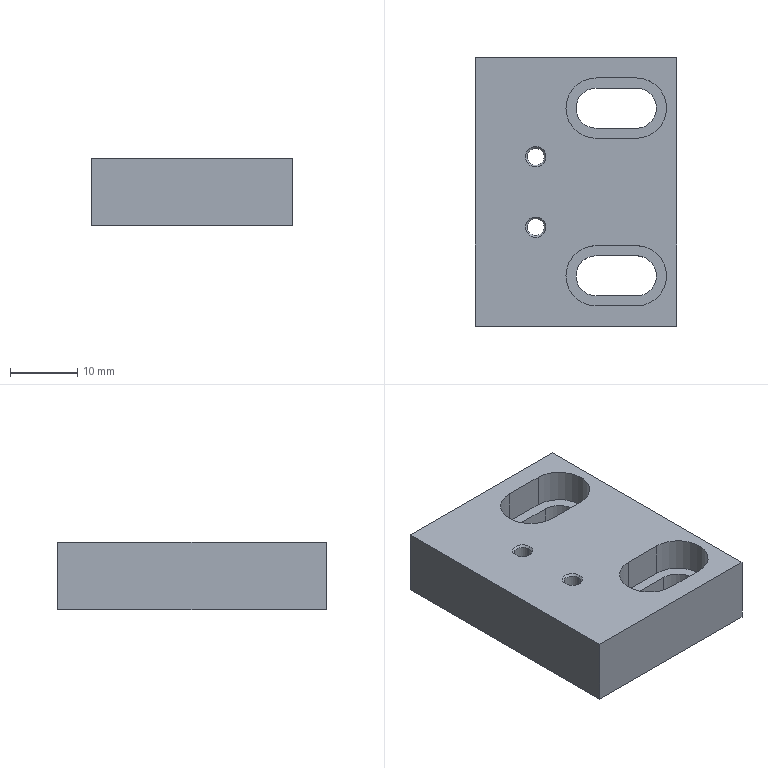Component | SolidWorks | PhotoelectricMount-1 | 1 solid | 36 faces | box 30 x 40 x 10 mm | volume 10082 mm3 | cylinder 16 | plane 16 | cone 4 | commonest cylinder face diameters 6 x6 9 x6 2.5 x4
STEP:
#1=CARTESIAN_POINT('',(-3.061,-2.53,-9.952));
#2=VERTEX_POINT('',#1);
#3=CARTESIAN_POINT('',(-3.159,-2.53,-9.952));
#4=VERTEX_POINT('',#3);
#5=CARTESIAN_POINT('',(-3.11,-2.53,-9.952));
#6=DIRECTION('',(-0.,0.,1.));
#7=DIRECTION('',(-1.,0.,0.));
#8=AXIS2_PLACEMENT_3D('',#5,#6,#7);
#9=CIRCLE('',#8,0.04921);
#10=EDGE_CURVE('',#2,#4,#9,.T.);
#11=ORIENTED_EDGE('',*,*,#10,.F.);
#12=CARTESIAN_POINT('',(-3.05,-2.53,-9.941));
#13=VERTEX_POINT('',#12);
#14=CARTESIAN_POINT('',(-3.061,-2.53,-9.952));
#15=DIRECTION('',(0.7071,-0.,0.7071));
#16=VECTOR('',#15,39.37);
#17=LINE('',#14,#16);
#18=EDGE_CURVE('',#2,#13,#17,.T.);
#19=ORIENTED_EDGE('',*,*,#18,.T.);
#20=CARTESIAN_POINT('',(-3.17,-2.53,-9.941));
#21=VERTEX_POINT('',#20);
#22=CARTESIAN_POINT('',(-3.11,-2.53,-9.941));
#23=DIRECTION('',(0.,0.,-1.));
#24=DIRECTION('',(-1.,0.,0.));
#25=AXIS2_PLACEMENT_3D('',#22,#23,#24);
#26=CIRCLE('',#25,0.06004);
#27=EDGE_CURVE('',#21,#13,#26,.T.);
#28=ORIENTED_EDGE('',*,*,#27,.F.);
#29=CARTESIAN_POINT('',(-3.159,-2.53,-9.952));
#30=DIRECTION('',(-0.7071,0.,0.7071));
#31=VECTOR('',#30,39.37);
#32=LINE('',#29,#31);
#33=EDGE_CURVE('',#4,#21,#32,.T.);
#34=ORIENTED_EDGE('',*,*,#33,.F.);
#35=EDGE_LOOP('',(#11,#19,#28,#34));
#36=FACE_OUTER_BOUND('',#35,.T.);
#37=CARTESIAN_POINT('',(-3.11,-2.53,-9.952));
#38=DIRECTION('',(-0.,0.,1.));
#39=DIRECTION('',(-1.,0.,0.));
#40=AXIS2_PLACEMENT_3D('',#37,#38,#39);
#41=CONICAL_SURFACE('',#40,0.04921,0.7854);
#42=ADVANCED_FACE('',(#36),#41,.F.);
#43=CARTESIAN_POINT('',(-3.061,-2.943,-9.952));
#44=VERTEX_POINT('',#43);
#45=CARTESIAN_POINT('',(-3.159,-2.943,-9.952));
#46=VERTEX_POINT('',#45);
#47=CARTESIAN_POINT('',(-3.11,-2.943,-9.952));
#48=DIRECTION('',(-0.,0.,1.));
#49=DIRECTION('',(-1.,0.,0.));
#50=AXIS2_PLACEMENT_3D('',#47,#48,#49);
#51=CIRCLE('',#50,0.04921);
#52=EDGE_CURVE('',#44,#46,#51,.T.);
#53=ORIENTED_EDGE('',*,*,#52,.F.);
#54=CARTESIAN_POINT('',(-3.05,-2.943,-9.941));
#55=VERTEX_POINT('',#54);
#56=CARTESIAN_POINT('',(-3.061,-2.943,-9.952));
#57=DIRECTION('',(0.7071,-0.,0.7071));
#58=VECTOR('',#57,39.37);
#59=LINE('',#56,#58);
#60=EDGE_CURVE('',#44,#55,#59,.T.);
#61=ORIENTED_EDGE('',*,*,#60,.T.);
#62=CARTESIAN_POINT('',(-3.17,-2.943,-9.941));
#63=VERTEX_POINT('',#62);
#64=CARTESIAN_POINT('',(-3.11,-2.943,-9.941));
#65=DIRECTION('',(0.,0.,-1.));
#66=DIRECTION('',(-1.,0.,0.));
#67=AXIS2_PLACEMENT_3D('',#64,#65,#66);
#68=CIRCLE('',#67,0.06004);
#69=EDGE_CURVE('',#63,#55,#68,.T.);
#70=ORIENTED_EDGE('',*,*,#69,.F.);
#71=CARTESIAN_POINT('',(-3.159,-2.943,-9.952));
#72=DIRECTION('',(-0.7071,0.,0.7071));
#73=VECTOR('',#72,39.37);
#74=LINE('',#71,#73);
#75=EDGE_CURVE('',#46,#63,#74,.T.);
#76=ORIENTED_EDGE('',*,*,#75,.F.);
#77=EDGE_LOOP('',(#53,#61,#70,#76));
#78=FACE_OUTER_BOUND('',#77,.T.);
#79=CARTESIAN_POINT('',(-3.11,-2.943,-9.952));
#80=DIRECTION('',(-0.,0.,1.));
#81=DIRECTION('',(-1.,0.,0.));
#82=AXIS2_PLACEMENT_3D('',#79,#80,#81);
#83=CONICAL_SURFACE('',#82,0.04921,0.7854);
#84=ADVANCED_FACE('',(#78),#83,.F.);
#85=CARTESIAN_POINT('',(-3.061,-2.53,-10.335));
#86=VERTEX_POINT('',#85);
#87=CARTESIAN_POINT('',(-3.159,-2.53,-10.335));
#88=VERTEX_POINT('',#87);
#89=CARTESIAN_POINT('',(-3.11,-2.53,-10.335));
#90=DIRECTION('',(-0.,0.,1.));
#91=DIRECTION('',(-1.,0.,0.));
#92=AXIS2_PLACEMENT_3D('',#89,#90,#91);
#93=CIRCLE('',#92,0.04921);
#94=EDGE_CURVE('',#86,#88,#93,.T.);
#95=ORIENTED_EDGE('',*,*,#94,.F.);
#96=CARTESIAN_POINT('',(-3.061,-2.53,-9.941));
#97=DIRECTION('',(-0.,0.,1.));
#98=VECTOR('',#97,39.37);
#99=LINE('',#96,#98);
#100=EDGE_CURVE('',#86,#2,#99,.T.);
#101=ORIENTED_EDGE('',*,*,#100,.T.);
#102=ORIENTED_EDGE('',*,*,#10,.T.);
#103=CARTESIAN_POINT('',(-3.159,-2.53,-9.941));
#104=DIRECTION('',(-0.,0.,1.));
#105=VECTOR('',#104,39.37);
#106=LINE('',#103,#105);
#107=EDGE_CURVE('',#88,#4,#106,.T.);
#108=ORIENTED_EDGE('',*,*,#107,.F.);
#109=EDGE_LOOP('',(#95,#101,#102,#108));
#110=FACE_OUTER_BOUND('',#109,.T.);
#111=CARTESIAN_POINT('',(-3.11,-2.53,-9.941));
#112=DIRECTION('',(-0.,0.,1.));
#113=DIRECTION('',(-1.,0.,0.));
#114=AXIS2_PLACEMENT_3D('',#111,#112,#113);
#115=CYLINDRICAL_SURFACE('',#114,0.04921);
#116=ADVANCED_FACE('',(#110),#115,.F.);
#117=CARTESIAN_POINT('',(-3.061,-2.943,-10.335));
#118=VERTEX_POINT('',#117);
#119=CARTESIAN_POINT('',(-3.159,-2.943,-10.335));
#120=VERTEX_POINT('',#119);
#121=CARTESIAN_POINT('',(-3.11,-2.943,-10.335));
#122=DIRECTION('',(-0.,0.,1.));
#123=DIRECTION('',(-1.,0.,0.));
#124=AXIS2_PLACEMENT_3D('',#121,#122,#123);
#125=CIRCLE('',#124,0.04921);
#126=EDGE_CURVE('',#118,#120,#125,.T.);
#127=ORIENTED_EDGE('',*,*,#126,.F.);
#128=CARTESIAN_POINT('',(-3.061,-2.943,-9.941));
#129=DIRECTION('',(-0.,0.,1.));
#130=VECTOR('',#129,39.37);
#131=LINE('',#128,#130);
#132=EDGE_CURVE('',#118,#44,#131,.T.);
#133=ORIENTED_EDGE('',*,*,#132,.T.);
#134=ORIENTED_EDGE('',*,*,#52,.T.);
#135=CARTESIAN_POINT('',(-3.159,-2.943,-9.941));
#136=DIRECTION('',(-0.,0.,1.));
#137=VECTOR('',#136,39.37);
#138=LINE('',#135,#137);
#139=EDGE_CURVE('',#120,#46,#138,.T.);
#140=ORIENTED_EDGE('',*,*,#139,.F.);
#141=EDGE_LOOP('',(#127,#133,#134,#140));
#142=FACE_OUTER_BOUND('',#141,.T.);
#143=CARTESIAN_POINT('',(-3.11,-2.943,-9.941));
#144=DIRECTION('',(-0.,0.,1.));
#145=DIRECTION('',(-1.,0.,0.));
#146=AXIS2_PLACEMENT_3D('',#143,#144,#145);
#147=CYLINDRICAL_SURFACE('',#146,0.04921);
#148=ADVANCED_FACE('',(#142),#147,.F.);
#149=CARTESIAN_POINT('',(-2.52,-2.362,-10.138));
#150=VERTEX_POINT('',#149);
#151=CARTESIAN_POINT('',(-2.402,-2.244,-10.138));
#152=VERTEX_POINT('',#151);
#153=CARTESIAN_POINT('',(-2.52,-2.244,-10.138));
#154=DIRECTION('',(-0.,0.,1.));
#155=DIRECTION('',(-1.,0.,0.));
#156=AXIS2_PLACEMENT_3D('',#153,#154,#155);
#157=CIRCLE('',#156,0.1181);
#158=EDGE_CURVE('',#150,#152,#157,.T.);
#159=ORIENTED_EDGE('',*,*,#158,.T.);
#160=CARTESIAN_POINT('',(-2.402,-2.244,-10.335));
#161=VERTEX_POINT('',#160);
#162=CARTESIAN_POINT('',(-2.402,-2.244,-9.941));
#163=DIRECTION('',(0.,0.,-1.));
#164=VECTOR('',#163,39.37);
#165=LINE('',#162,#164);
#166=EDGE_CURVE('',#152,#161,#165,.T.);
#167=ORIENTED_EDGE('',*,*,#166,.T.);
#168=CARTESIAN_POINT('',(-2.52,-2.362,-10.335));
#169=VERTEX_POINT('',#168);
#170=CARTESIAN_POINT('',(-2.52,-2.244,-10.335));
#171=DIRECTION('',(0.,0.,-1.));
#172=DIRECTION('',(1.,0.,0.));
#173=AXIS2_PLACEMENT_3D('',#170,#171,#172);
#174=CIRCLE('',#173,0.1181);
#175=EDGE_CURVE('',#161,#169,#174,.T.);
#176=ORIENTED_EDGE('',*,*,#175,.T.);
#177=CARTESIAN_POINT('',(-2.52,-2.362,-9.941));
#178=DIRECTION('',(0.,0.,-1.));
#179=VECTOR('',#178,39.37);
#180=LINE('',#177,#179);
#181=EDGE_CURVE('',#150,#169,#180,.T.);
#182=ORIENTED_EDGE('',*,*,#181,.F.);
#183=EDGE_LOOP('',(#159,#167,#176,#182));
#184=FACE_OUTER_BOUND('',#183,.T.);
#185=CARTESIAN_POINT('',(-2.52,-2.244,-9.941));
#186=DIRECTION('',(0.,0.,-1.));
#187=DIRECTION('',(1.,0.,0.));
#188=AXIS2_PLACEMENT_3D('',#185,#186,#187);
#189=CYLINDRICAL_SURFACE('',#188,0.1181);
#190=ADVANCED_FACE('',(#184),#189,.F.);
#191=CARTESIAN_POINT('',(-2.933,-2.244,-10.138));
#192=VERTEX_POINT('',#191);
#193=CARTESIAN_POINT('',(-2.756,-2.421,-10.138));
#194=VERTEX_POINT('',#193);
#195=CARTESIAN_POINT('',(-2.756,-2.244,-10.138));
#196=DIRECTION('',(-0.,0.,1.));
#197=DIRECTION('',(-1.,0.,0.));
#198=AXIS2_PLACEMENT_3D('',#195,#196,#197);
#199=CIRCLE('',#198,0.1772);
#200=EDGE_CURVE('',#192,#194,#199,.T.);
#201=ORIENTED_EDGE('',*,*,#200,.F.);
#202=CARTESIAN_POINT('',(-2.933,-2.244,-9.941));
#203=VERTEX_POINT('',#202);
#204=CARTESIAN_POINT('',(-2.933,-2.244,-10.138));
#205=DIRECTION('',(-0.,0.,1.));
#206=VECTOR('',#205,39.37);
#207=LINE('',#204,#206);
#208=EDGE_CURVE('',#192,#203,#207,.T.);
#209=ORIENTED_EDGE('',*,*,#208,.T.);
#210=CARTESIAN_POINT('',(-2.756,-2.421,-9.941));
#211=VERTEX_POINT('',#210);
#212=CARTESIAN_POINT('',(-2.756,-2.244,-9.941));
#213=DIRECTION('',(-0.,0.,1.));
#214=DIRECTION('',(-1.,0.,0.));
#215=AXIS2_PLACEMENT_3D('',#212,#213,#214);
#216=CIRCLE('',#215,0.1772);
#217=EDGE_CURVE('',#203,#211,#216,.T.);
#218=ORIENTED_EDGE('',*,*,#217,.T.);
#219=CARTESIAN_POINT('',(-2.756,-2.421,-10.138));
#220=DIRECTION('',(-0.,0.,1.));
#221=VECTOR('',#220,39.37);
#222=LINE('',#219,#221);
#223=EDGE_CURVE('',#194,#211,#222,.T.);
#224=ORIENTED_EDGE('',*,*,#223,.F.);
#225=EDGE_LOOP('',(#201,#209,#218,#224));
#226=FACE_OUTER_BOUND('',#225,.T.);
#227=CARTESIAN_POINT('',(-2.756,-2.244,-10.138));
#228=DIRECTION('',(-0.,0.,1.));
#229=DIRECTION('',(-1.,0.,0.));
#230=AXIS2_PLACEMENT_3D('',#227,#228,#229);
#231=CYLINDRICAL_SURFACE('',#230,0.1772);
#232=ADVANCED_FACE('',(#226),#231,.F.);
#233=CARTESIAN_POINT('',(-2.52,-3.346,-10.138));
#234=VERTEX_POINT('',#233);
#235=CARTESIAN_POINT('',(-2.402,-3.228,-10.138));
#236=VERTEX_POINT('',#235);
#237=CARTESIAN_POINT('',(-2.52,-3.228,-10.138));
#238=DIRECTION('',(-0.,0.,1.));
#239=DIRECTION('',(-1.,0.,0.));
#240=AXIS2_PLACEMENT_3D('',#237,#238,#239);
#241=CIRCLE('',#240,0.1181);
#242=EDGE_CURVE('',#234,#236,#241,.T.);
#243=ORIENTED_EDGE('',*,*,#242,.T.);
#244=CARTESIAN_POINT('',(-2.402,-3.228,-10.335));
#245=VERTEX_POINT('',#244);
#246=CARTESIAN_POINT('',(-2.402,-3.228,-9.941));
#247=DIRECTION('',(0.,0.,-1.));
#248=VECTOR('',#247,39.37);
#249=LINE('',#246,#248);
#250=EDGE_CURVE('',#236,#245,#249,.T.);
#251=ORIENTED_EDGE('',*,*,#250,.T.);
#252=CARTESIAN_POINT('',(-2.52,-3.346,-10.335));
#253=VERTEX_POINT('',#252);
#254=CARTESIAN_POINT('',(-2.52,-3.228,-10.335));
#255=DIRECTION('',(0.,0.,-1.));
#256=DIRECTION('',(1.,0.,0.));
#257=AXIS2_PLACEMENT_3D('',#254,#255,#256);
#258=CIRCLE('',#257,0.1181);
#259=EDGE_CURVE('',#245,#253,#258,.T.);
#260=ORIENTED_EDGE('',*,*,#259,.T.);
#261=CARTESIAN_POINT('',(-2.52,-3.346,-9.941));
#262=DIRECTION('',(0.,0.,-1.));
#263=VECTOR('',#262,39.37);
#264=LINE('',#261,#263);
#265=EDGE_CURVE('',#234,#253,#264,.T.);
#266=ORIENTED_EDGE('',*,*,#265,.F.);
#267=EDGE_LOOP('',(#243,#251,#260,#266));
#268=FACE_OUTER_BOUND('',#267,.T.);
#269=CARTESIAN_POINT('',(-2.52,-3.228,-9.941));
#270=DIRECTION('',(0.,0.,-1.));
#271=DIRECTION('',(1.,0.,0.));
#272=AXIS2_PLACEMENT_3D('',#269,#270,#271);
#273=CYLINDRICAL_SURFACE('',#272,0.1181);
#274=ADVANCED_FACE('',(#268),#273,.F.);
#275=CARTESIAN_POINT('',(-2.933,-3.228,-10.138));
#276=VERTEX_POINT('',#275);
#277=CARTESIAN_POINT('',(-2.756,-3.406,-10.138));
#278=VERTEX_POINT('',#277);
#279=CARTESIAN_POINT('',(-2.756,-3.228,-10.138));
#280=DIRECTION('',(-0.,0.,1.));
#281=DIRECTION('',(-1.,0.,0.));
#282=AXIS2_PLACEMENT_3D('',#279,#280,#281);
#283=CIRCLE('',#282,0.1772);
#284=EDGE_CURVE('',#276,#278,#283,.T.);
#285=ORIENTED_EDGE('',*,*,#284,.F.);
#286=CARTESIAN_POINT('',(-2.933,-3.228,-9.941));
#287=VERTEX_POINT('',#286);
#288=CARTESIAN_POINT('',(-2.933,-3.228,-10.138));
#289=DIRECTION('',(-0.,0.,1.));
#290=VECTOR('',#289,39.37);
#291=LINE('',#288,#290);
#292=EDGE_CURVE('',#276,#287,#291,.T.);
#293=ORIENTED_EDGE('',*,*,#292,.T.);
#294=CARTESIAN_POINT('',(-2.756,-3.406,-9.941));
#295=VERTEX_POINT('',#294);
#296=CARTESIAN_POINT('',(-2.756,-3.228,-9.941));
#297=DIRECTION('',(-0.,0.,1.));
#298=DIRECTION('',(-1.,0.,0.));
#299=AXIS2_PLACEMENT_3D('',#296,#297,#298);
#300=CIRCLE('',#299,0.1772);
#301=EDGE_CURVE('',#287,#295,#300,.T.);
#302=ORIENTED_EDGE('',*,*,#301,.T.);
#303=CARTESIAN_POINT('',(-2.756,-3.406,-10.138));
#304=DIRECTION('',(-0.,0.,1.));
#305=VECTOR('',#304,39.37);
#306=LINE('',#303,#305);
#307=EDGE_CURVE('',#278,#295,#306,.T.);
#308=ORIENTED_EDGE('',*,*,#307,.F.);
#309=EDGE_LOOP('',(#285,#293,#302,#308));
#310=FACE_OUTER_BOUND('',#309,.T.);
#311=CARTESIAN_POINT('',(-2.756,-3.228,-10.138));
#312=DIRECTION('',(-0.,0.,1.));
#313=DIRECTION('',(-1.,0.,0.));
#314=AXIS2_PLACEMENT_3D('',#311,#312,#313);
#315=CYLINDRICAL_SURFACE('',#314,0.1772);
#316=ADVANCED_FACE('',(#310),#315,.F.);
#317=CARTESIAN_POINT('',(-3.465,-3.524,-9.941));
#318=VERTEX_POINT('',#317);
#319=CARTESIAN_POINT('',(-2.283,-3.524,-9.941));
#320=VERTEX_POINT('',#319);
#321=CARTESIAN_POINT('',(-3.465,-3.524,-9.941));
#322=DIRECTION('',(1.,-0.,0.));
#323=VECTOR('',#322,39.37);
#324=LINE('',#321,#323);
#325=EDGE_CURVE('',#318,#320,#324,.T.);
#326=ORIENTED_EDGE('',*,*,#325,.F.);
#327=CARTESIAN_POINT('',(-3.465,-3.524,-10.335));
#328=VERTEX_POINT('',#327);
#329=CARTESIAN_POINT('',(-3.465,-3.524,-10.335));
#330=DIRECTION('',(-0.,0.,1.));
#331=VECTOR('',#330,39.37);
#332=LINE('',#329,#331);
#333=EDGE_CURVE('',#328,#318,#332,.T.);
#334=ORIENTED_EDGE('',*,*,#333,.F.);
#335=CARTESIAN_POINT('',(-2.283,-3.524,-10.335));
#336=VERTEX_POINT('',#335);
#337=CARTESIAN_POINT('',(-3.465,-3.524,-10.335));
#338=DIRECTION('',(1.,-0.,0.));
#339=VECTOR('',#338,39.37);
#340=LINE('',#337,#339);
#341=EDGE_CURVE('',#328,#336,#340,.T.);
#342=ORIENTED_EDGE('',*,*,#341,.T.);
#343=CARTESIAN_POINT('',(-2.283,-3.524,-10.335));
#344=DIRECTION('',(-0.,0.,1.));
#345=VECTOR('',#344,39.37);
#346=LINE('',#343,#345);
#347=EDGE_CURVE('',#336,#320,#346,.T.);
#348=ORIENTED_EDGE('',*,*,#347,.T.);
#349=EDGE_LOOP('',(#326,#334,#342,#348));
#350=FACE_OUTER_BOUND('',#349,.T.);
#351=CARTESIAN_POINT('',(-3.465,-3.524,-10.335));
#352=DIRECTION('',(-0.,-1.,-0.));
#353=DIRECTION('',(-0.,0.,1.));
#354=AXIS2_PLACEMENT_3D('',#351,#352,#353);
#355=PLANE('',#354);
#356=ADVANCED_FACE('',(#350),#355,.T.);
#357=CARTESIAN_POINT('',(-3.465,-1.949,-9.941));
#358=VERTEX_POINT('',#357);
#359=CARTESIAN_POINT('',(-3.465,-1.949,-9.941));
#360=DIRECTION('',(-0.,-1.,-0.));
#361=VECTOR('',#360,39.37);
#362=LINE('',#359,#361);
#363=EDGE_CURVE('',#358,#318,#362,.T.);
#364=ORIENTED_EDGE('',*,*,#363,.F.);
#365=CARTESIAN_POINT('',(-3.465,-1.949,-10.335));
#366=VERTEX_POINT('',#365);
#367=CARTESIAN_POINT('',(-3.465,-1.949,-10.335));
#368=DIRECTION('',(-0.,0.,1.));
#369=VECTOR('',#368,39.37);
#370=LINE('',#367,#369);
#371=EDGE_CURVE('',#366,#358,#370,.T.);
#372=ORIENTED_EDGE('',*,*,#371,.F.);
#373=CARTESIAN_POINT('',(-3.465,-1.949,-10.335));
#374=DIRECTION('',(-0.,-1.,-0.));
#375=VECTOR('',#374,39.37);
#376=LINE('',#373,#375);
#377=EDGE_CURVE('',#366,#328,#376,.T.);
#378=ORIENTED_EDGE('',*,*,#377,.T.);
#379=ORIENTED_EDGE('',*,*,#333,.T.);
#380=EDGE_LOOP('',(#364,#372,#378,#379));
#381=FACE_OUTER_BOUND('',#380,.T.);
#382=CARTESIAN_POINT('',(-3.465,-1.949,-10.335));
#383=DIRECTION('',(-1.,0.,-0.));
#384=DIRECTION('',(0.,0.,-1.));
#385=AXIS2_PLACEMENT_3D('',#382,#383,#384);
#386=PLANE('',#385);
#387=ADVANCED_FACE('',(#381),#386,.T.);
#388=CARTESIAN_POINT('',(-2.283,-1.949,-9.941));
#389=VERTEX_POINT('',#388);
#390=CARTESIAN_POINT('',(-2.283,-1.949,-9.941));
#391=DIRECTION('',(-1.,0.,-0.));
#392=VECTOR('',#391,39.37);
#393=LINE('',#390,#392);
#394=EDGE_CURVE('',#389,#358,#393,.T.);
#395=ORIENTED_EDGE('',*,*,#394,.F.);
#396=CARTESIAN_POINT('',(-2.283,-1.949,-10.335));
#397=VERTEX_POINT('',#396);
#398=CARTESIAN_POINT('',(-2.283,-1.949,-10.335));
#399=DIRECTION('',(-0.,0.,1.));
#400=VECTOR('',#399,39.37);
#401=LINE('',#398,#400);
#402=EDGE_CURVE('',#397,#389,#401,.T.);
#403=ORIENTED_EDGE('',*,*,#402,.F.);
#404=CARTESIAN_POINT('',(-2.283,-1.949,-10.335));
#405=DIRECTION('',(-1.,0.,-0.));
#406=VECTOR('',#405,39.37);
#407=LINE('',#404,#406);
#408=EDGE_CURVE('',#397,#366,#407,.T.);
#409=ORIENTED_EDGE('',*,*,#408,.T.);
#410=ORIENTED_EDGE('',*,*,#371,.T.);
#411=EDGE_LOOP('',(#395,#403,#409,#410));
#412=FACE_OUTER_BOUND('',#411,.T.);
#413=CARTESIAN_POINT('',(-2.283,-1.949,-10.335));
#414=DIRECTION('',(0.,1.,0.));
#415=DIRECTION('',(0.,0.,-1.));
#416=AXIS2_PLACEMENT_3D('',#413,#414,#415);
#417=PLANE('',#416);
#418=ADVANCED_FACE('',(#412),#417,.T.);
#419=CARTESIAN_POINT('',(-2.283,-3.524,-9.941));
#420=DIRECTION('',(0.,1.,0.));
#421=VECTOR('',#420,39.37);
#422=LINE('',#419,#421);
#423=EDGE_CURVE('',#320,#389,#422,.T.);
#424=ORIENTED_EDGE('',*,*,#423,.F.);
#425=ORIENTED_EDGE('',*,*,#347,.F.);
#426=CARTESIAN_POINT('',(-2.283,-3.524,-10.335));
#427=DIRECTION('',(0.,1.,0.));
#428=VECTOR('',#427,39.37);
#429=LINE('',#426,#428);
#430=EDGE_CURVE('',#336,#397,#429,.T.);
#431=ORIENTED_EDGE('',*,*,#430,.T.);
#432=ORIENTED_EDGE('',*,*,#402,.T.);
#433=EDGE_LOOP('',(#424,#425,#431,#432));
#434=FACE_OUTER_BOUND('',#433,.T.);
#435=CARTESIAN_POINT('',(-2.283,-3.524,-10.335));
#436=DIRECTION('',(1.,-0.,0.));
#437=DIRECTION('',(-0.,0.,1.));
#438=AXIS2_PLACEMENT_3D('',#435,#436,#437);
#439=PLANE('',#438);
#440=ADVANCED_FACE('',(#434),#439,.T.);
#441=CARTESIAN_POINT('',(-3.11,-2.53,-10.335));
#442=DIRECTION('',(-0.,0.,1.));
#443=DIRECTION('',(-1.,0.,0.));
#444=AXIS2_PLACEMENT_3D('',#441,#442,#443);
#445=CIRCLE('',#444,0.04921);
#446=EDGE_CURVE('',#88,#86,#445,.T.);
#447=ORIENTED_EDGE('',*,*,#446,.T.);
#448=ORIENTED_EDGE('',*,*,#94,.T.);
#449=EDGE_LOOP('',(#447,#448));
#450=FACE_BOUND('',#449,.T.);
#451=CARTESIAN_POINT('',(-3.11,-2.943,-10.335));
#452=DIRECTION('',(-0.,0.,1.));
#453=DIRECTION('',(-1.,0.,0.));
#454=AXIS2_PLACEMENT_3D('',#451,#452,#453);
#455=CIRCLE('',#454,0.04921);
#456=EDGE_CURVE('',#120,#118,#455,.T.);
#457=ORIENTED_EDGE('',*,*,#456,.T.);
#458=ORIENTED_EDGE('',*,*,#126,.T.);
#459=EDGE_LOOP('',(#457,#458));
#460=FACE_BOUND('',#459,.T.);
#461=CARTESIAN_POINT('',(-2.756,-2.362,-10.335));
#462=VERTEX_POINT('',#461);
#463=CARTESIAN_POINT('',(-2.52,-2.362,-10.335));
#464=DIRECTION('',(-1.,0.,-0.));
#465=VECTOR('',#464,39.37);
#466=LINE('',#463,#465);
#467=EDGE_CURVE('',#169,#462,#466,.T.);
#468=ORIENTED_EDGE('',*,*,#467,.F.);
#469=ORIENTED_EDGE('',*,*,#175,.F.);
#470=CARTESIAN_POINT('',(-2.52,-2.126,-10.335));
#471=VERTEX_POINT('',#470);
#472=CARTESIAN_POINT('',(-2.52,-2.244,-10.335));
#473=DIRECTION('',(0.,0.,-1.));
#474=DIRECTION('',(1.,0.,0.));
#475=AXIS2_PLACEMENT_3D('',#472,#473,#474);
#476=CIRCLE('',#475,0.1181);
#477=EDGE_CURVE('',#471,#161,#476,.T.);
#478=ORIENTED_EDGE('',*,*,#477,.F.);
#479=CARTESIAN_POINT('',(-2.756,-2.126,-10.335));
#480=VERTEX_POINT('',#479);
#481=CARTESIAN_POINT('',(-2.756,-2.126,-10.335));
#482=DIRECTION('',(1.,-0.,0.));
#483=VECTOR('',#482,39.37);
#484=LINE('',#481,#483);
#485=EDGE_CURVE('',#480,#471,#484,.T.);
#486=ORIENTED_EDGE('',*,*,#485,.F.);
#487=CARTESIAN_POINT('',(-2.756,-2.244,-10.335));
#488=DIRECTION('',(0.,0.,-1.));
#489=DIRECTION('',(1.,0.,0.));
#490=AXIS2_PLACEMENT_3D('',#487,#488,#489);
#491=CIRCLE('',#490,0.1181);
#492=EDGE_CURVE('',#462,#480,#491,.T.);
#493=ORIENTED_EDGE('',*,*,#492,.F.);
#494=EDGE_LOOP('',(#468,#469,#478,#486,#493));
#495=FACE_BOUND('',#494,.T.);
#496=CARTESIAN_POINT('',(-2.756,-3.346,-10.335));
#497=VERTEX_POINT('',#496);
#498=CARTESIAN_POINT('',(-2.52,-3.346,-10.335));
#499=DIRECTION('',(-1.,0.,-0.));
#500=VECTOR('',#499,39.37);
#501=LINE('',#498,#500);
#502=EDGE_CURVE('',#253,#497,#501,.T.);
#503=ORIENTED_EDGE('',*,*,#502,.F.);
#504=ORIENTED_EDGE('',*,*,#259,.F.);
#505=CARTESIAN_POINT('',(-2.52,-3.11,-10.335));
#506=VERTEX_POINT('',#505);
#507=CARTESIAN_POINT('',(-2.52,-3.228,-10.335));
#508=DIRECTION('',(0.,0.,-1.));
#509=DIRECTION('',(1.,0.,0.));
#510=AXIS2_PLACEMENT_3D('',#507,#508,#509);
#511=CIRCLE('',#510,0.1181);
#512=EDGE_CURVE('',#506,#245,#511,.T.);
#513=ORIENTED_EDGE('',*,*,#512,.F.);
#514=CARTESIAN_POINT('',(-2.756,-3.11,-10.335));
#515=VERTEX_POINT('',#514);
#516=CARTESIAN_POINT('',(-2.756,-3.11,-10.335));
#517=DIRECTION('',(1.,-0.,0.));
#518=VECTOR('',#517,39.37);
#519=LINE('',#516,#518);
#520=EDGE_CURVE('',#515,#506,#519,.T.);
#521=ORIENTED_EDGE('',*,*,#520,.F.);
#522=CARTESIAN_POINT('',(-2.756,-3.228,-10.335));
#523=DIRECTION('',(0.,0.,-1.));
#524=DIRECTION('',(1.,0.,0.));
#525=AXIS2_PLACEMENT_3D('',#522,#523,#524);
#526=CIRCLE('',#525,0.1181);
#527=EDGE_CURVE('',#497,#515,#526,.T.);
#528=ORIENTED_EDGE('',*,*,#527,.F.);
#529=EDGE_LOOP('',(#503,#504,#513,#521,#528));
#530=FACE_BOUND('',#529,.T.);
#531=ORIENTED_EDGE('',*,*,#341,.F.);
#532=ORIENTED_EDGE('',*,*,#377,.F.);
#533=ORIENTED_EDGE('',*,*,#408,.F.);
#534=ORIENTED_EDGE('',*,*,#430,.F.);
#535=EDGE_LOOP('',(#531,#532,#533,#534));
#536=FACE_OUTER_BOUND('',#535,.T.);
#537=CARTESIAN_POINT('',(-2.874,-2.736,-10.335));
#538=DIRECTION('',(-0.,0.,1.));
#539=DIRECTION('',(-1.,0.,-0.));
#540=AXIS2_PLACEMENT_3D('',#537,#538,#539);
#541=PLANE('',#540);
#542=ADVANCED_FACE('',(#450,#460,#495,#530,#536),#541,.F.);
#543=ORIENTED_EDGE('',*,*,#69,.T.);
#544=CARTESIAN_POINT('',(-3.11,-2.943,-9.941));
#545=DIRECTION('',(0.,0.,-1.));
#546=DIRECTION('',(-1.,0.,0.));
#547=AXIS2_PLACEMENT_3D('',#544,#545,#546);
#548=CIRCLE('',#547,0.06004);
#549=EDGE_CURVE('',#55,#63,#548,.T.);
#550=ORIENTED_EDGE('',*,*,#549,.T.);
#551=EDGE_LOOP('',(#543,#550));
#552=FACE_BOUND('',#551,.T.);
#553=ORIENTED_EDGE('',*,*,#27,.T.);
#554=CARTESIAN_POINT('',(-3.11,-2.53,-9.941));
#555=DIRECTION('',(0.,0.,-1.));
#556=DIRECTION('',(-1.,0.,0.));
#557=AXIS2_PLACEMENT_3D('',#554,#555,#556);
#558=CIRCLE('',#557,0.06004);
#559=EDGE_CURVE('',#13,#21,#558,.T.);
#560=ORIENTED_EDGE('',*,*,#559,.T.);
#561=EDGE_LOOP('',(#553,#560));
#562=FACE_BOUND('',#561,.T.);
#563=CARTESIAN_POINT('',(-2.756,-2.067,-9.941));
#564=VERTEX_POINT('',#563);
#565=CARTESIAN_POINT('',(-2.756,-2.244,-9.941));
#566=DIRECTION('',(-0.,0.,1.));
#567=DIRECTION('',(-1.,0.,0.));
#568=AXIS2_PLACEMENT_3D('',#565,#566,#567);
#569=CIRCLE('',#568,0.1772);
#570=EDGE_CURVE('',#564,#203,#569,.T.);
#571=ORIENTED_EDGE('',*,*,#570,.F.);
#572=CARTESIAN_POINT('',(-2.52,-2.067,-9.941));
#573=VERTEX_POINT('',#572);
#574=CARTESIAN_POINT('',(-2.52,-2.067,-9.941));
#575=DIRECTION('',(-1.,0.,-0.));
#576=VECTOR('',#575,39.37);
#577=LINE('',#574,#576);
#578=EDGE_CURVE('',#573,#564,#577,.T.);
#579=ORIENTED_EDGE('',*,*,#578,.F.);
#580=CARTESIAN_POINT('',(-2.52,-2.421,-9.941));
#581=VERTEX_POINT('',#580);
#582=CARTESIAN_POINT('',(-2.52,-2.244,-9.941));
#583=DIRECTION('',(-0.,0.,1.));
#584=DIRECTION('',(-1.,0.,0.));
#585=AXIS2_PLACEMENT_3D('',#582,#583,#584);
#586=CIRCLE('',#585,0.1772);
#587=EDGE_CURVE('',#581,#573,#586,.T.);
#588=ORIENTED_EDGE('',*,*,#587,.F.);
#589=CARTESIAN_POINT('',(-2.756,-2.421,-9.941));
#590=DIRECTION('',(1.,-0.,0.));
#591=VECTOR('',#590,39.37);
#592=LINE('',#589,#591);
#593=EDGE_CURVE('',#211,#581,#592,.T.);
#594=ORIENTED_EDGE('',*,*,#593,.F.);
#595=ORIENTED_EDGE('',*,*,#217,.F.);
#596=EDGE_LOOP('',(#571,#579,#588,#594,#595));
#597=FACE_BOUND('',#596,.T.);
#598=CARTESIAN_POINT('',(-2.756,-3.051,-9.941));
#599=VERTEX_POINT('',#598);
#600=CARTESIAN_POINT('',(-2.756,-3.228,-9.941));
#601=DIRECTION('',(-0.,0.,1.));
#602=DIRECTION('',(-1.,0.,0.));
#603=AXIS2_PLACEMENT_3D('',#600,#601,#602);
#604=CIRCLE('',#603,0.1772);
#605=EDGE_CURVE('',#599,#287,#604,.T.);
#606=ORIENTED_EDGE('',*,*,#605,.F.);
#607=CARTESIAN_POINT('',(-2.52,-3.051,-9.941));
#608=VERTEX_POINT('',#607);
#609=CARTESIAN_POINT('',(-2.52,-3.051,-9.941));
#610=DIRECTION('',(-1.,0.,-0.));
#611=VECTOR('',#610,39.37);
#612=LINE('',#609,#611);
#613=EDGE_CURVE('',#608,#599,#612,.T.);
#614=ORIENTED_EDGE('',*,*,#613,.F.);
#615=CARTESIAN_POINT('',(-2.52,-3.406,-9.941));
#616=VERTEX_POINT('',#615);
#617=CARTESIAN_POINT('',(-2.52,-3.228,-9.941));
#618=DIRECTION('',(-0.,0.,1.));
#619=DIRECTION('',(-1.,0.,0.));
#620=AXIS2_PLACEMENT_3D('',#617,#618,#619);
#621=CIRCLE('',#620,0.1772);
#622=EDGE_CURVE('',#616,#608,#621,.T.);
#623=ORIENTED_EDGE('',*,*,#622,.F.);
#624=CARTESIAN_POINT('',(-2.756,-3.406,-9.941));
#625=DIRECTION('',(1.,-0.,0.));
#626=VECTOR('',#625,39.37);
#627=LINE('',#624,#626);
#628=EDGE_CURVE('',#295,#616,#627,.T.);
#629=ORIENTED_EDGE('',*,*,#628,.F.);
#630=ORIENTED_EDGE('',*,*,#301,.F.);
#631=EDGE_LOOP('',(#606,#614,#623,#629,#630));
#632=FACE_BOUND('',#631,.T.);
#633=ORIENTED_EDGE('',*,*,#325,.T.);
#634=ORIENTED_EDGE('',*,*,#423,.T.);
#635=ORIENTED_EDGE('',*,*,#394,.T.);
#636=ORIENTED_EDGE('',*,*,#363,.T.);
#637=EDGE_LOOP('',(#633,#634,#635,#636));
#638=FACE_OUTER_BOUND('',#637,.T.);
#639=CARTESIAN_POINT('',(-2.874,-2.736,-9.941));
#640=DIRECTION('',(-0.,0.,1.));
#641=DIRECTION('',(-1.,0.,-0.));
#642=AXIS2_PLACEMENT_3D('',#639,#640,#641);
#643=PLANE('',#642);
#644=ADVANCED_FACE('',(#552,#562,#597,#632,#638),#643,.T.);
#645=ORIENTED_EDGE('',*,*,#292,.F.);
#646=CARTESIAN_POINT('',(-2.756,-3.051,-10.138));
#647=VERTEX_POINT('',#646);
#648=CARTESIAN_POINT('',(-2.756,-3.228,-10.138));
#649=DIRECTION('',(-0.,0.,1.));
#650=DIRECTION('',(-1.,0.,0.));
#651=AXIS2_PLACEMENT_3D('',#648,#649,#650);
#652=CIRCLE('',#651,0.1772);
#653=EDGE_CURVE('',#647,#276,#652,.T.);
#654=ORIENTED_EDGE('',*,*,#653,.F.);
#655=CARTESIAN_POINT('',(-2.756,-3.051,-10.138));
#656=DIRECTION('',(-0.,0.,1.));
#657=VECTOR('',#656,39.37);
#658=LINE('',#655,#657);
#659=EDGE_CURVE('',#647,#599,#658,.T.);
#660=ORIENTED_EDGE('',*,*,#659,.T.);
#661=ORIENTED_EDGE('',*,*,#605,.T.);
#662=EDGE_LOOP('',(#645,#654,#660,#661));
#663=FACE_OUTER_BOUND('',#662,.T.);
#664=CARTESIAN_POINT('',(-2.756,-3.228,-10.138));
#665=DIRECTION('',(-0.,0.,1.));
#666=DIRECTION('',(-1.,0.,0.));
#667=AXIS2_PLACEMENT_3D('',#664,#665,#666);
#668=CYLINDRICAL_SURFACE('',#667,0.1772);
#669=ADVANCED_FACE('',(#663),#668,.F.);
#670=ORIENTED_EDGE('',*,*,#613,.T.);
#671=ORIENTED_EDGE('',*,*,#659,.F.);
#672=CARTESIAN_POINT('',(-2.52,-3.051,-10.138));
#673=VERTEX_POINT('',#672);
#674=CARTESIAN_POINT('',(-2.52,-3.051,-10.138));
#675=DIRECTION('',(-1.,0.,-0.));
#676=VECTOR('',#675,39.37);
#677=LINE('',#674,#676);
#678=EDGE_CURVE('',#673,#647,#677,.T.);
#679=ORIENTED_EDGE('',*,*,#678,.F.);
#680=CARTESIAN_POINT('',(-2.52,-3.051,-10.138));
#681=DIRECTION('',(-0.,0.,1.));
#682=VECTOR('',#681,39.37);
#683=LINE('',#680,#682);
#684=EDGE_CURVE('',#673,#608,#683,.T.);
#685=ORIENTED_EDGE('',*,*,#684,.T.);
#686=EDGE_LOOP('',(#670,#671,#679,#685));
#687=FACE_OUTER_BOUND('',#686,.T.);
#688=CARTESIAN_POINT('',(-2.52,-3.051,-10.138));
#689=DIRECTION('',(0.,1.,0.));
#690=DIRECTION('',(0.,0.,-1.));
#691=AXIS2_PLACEMENT_3D('',#688,#689,#690);
#692=PLANE('',#691);
#693=ADVANCED_FACE('',(#687),#692,.F.);
#694=ORIENTED_EDGE('',*,*,#622,.T.);
#695=ORIENTED_EDGE('',*,*,#684,.F.);
#696=CARTESIAN_POINT('',(-2.52,-3.406,-10.138));
#697=VERTEX_POINT('',#696);
#698=CARTESIAN_POINT('',(-2.52,-3.228,-10.138));
#699=DIRECTION('',(-0.,0.,1.));
#700=DIRECTION('',(-1.,0.,0.));
#701=AXIS2_PLACEMENT_3D('',#698,#699,#700);
#702=CIRCLE('',#701,0.1772);
#703=EDGE_CURVE('',#697,#673,#702,.T.);
#704=ORIENTED_EDGE('',*,*,#703,.F.);
#705=CARTESIAN_POINT('',(-2.52,-3.406,-10.138));
#706=DIRECTION('',(-0.,0.,1.));
#707=VECTOR('',#706,39.37);
#708=LINE('',#705,#707);
#709=EDGE_CURVE('',#697,#616,#708,.T.);
#710=ORIENTED_EDGE('',*,*,#709,.T.);
#711=EDGE_LOOP('',(#694,#695,#704,#710));
#712=FACE_OUTER_BOUND('',#711,.T.);
#713=CARTESIAN_POINT('',(-2.52,-3.228,-10.138));
#714=DIRECTION('',(-0.,0.,1.));
#715=DIRECTION('',(-1.,0.,0.));
#716=AXIS2_PLACEMENT_3D('',#713,#714,#715);
#717=CYLINDRICAL_SURFACE('',#716,0.1772);
#718=ADVANCED_FACE('',(#712),#717,.F.);
#719=ORIENTED_EDGE('',*,*,#628,.T.);
#720=ORIENTED_EDGE('',*,*,#709,.F.);
#721=CARTESIAN_POINT('',(-2.756,-3.406,-10.138));
#722=DIRECTION('',(1.,-0.,0.));
#723=VECTOR('',#722,39.37);
#724=LINE('',#721,#723);
#725=EDGE_CURVE('',#278,#697,#724,.T.);
#726=ORIENTED_EDGE('',*,*,#725,.F.);
#727=ORIENTED_EDGE('',*,*,#307,.T.);
#728=EDGE_LOOP('',(#719,#720,#726,#727));
#729=FACE_OUTER_BOUND('',#728,.T.);
#730=CARTESIAN_POINT('',(-2.756,-3.406,-10.138));
#731=DIRECTION('',(-0.,-1.,-0.));
#732=DIRECTION('',(-0.,0.,1.));
#733=AXIS2_PLACEMENT_3D('',#730,#731,#732);
#734=PLANE('',#733);
#735=ADVANCED_FACE('',(#729),#734,.F.);
#736=ORIENTED_EDGE('',*,*,#242,.F.);
#737=CARTESIAN_POINT('',(-2.756,-3.346,-10.138));
#738=VERTEX_POINT('',#737);
#739=CARTESIAN_POINT('',(-2.756,-3.346,-10.138));
#740=DIRECTION('',(1.,-0.,0.));
#741=VECTOR('',#740,39.37);
#742=LINE('',#739,#741);
#743=EDGE_CURVE('',#738,#234,#742,.T.);
#744=ORIENTED_EDGE('',*,*,#743,.F.);
#745=CARTESIAN_POINT('',(-2.756,-3.11,-10.138));
#746=VERTEX_POINT('',#745);
#747=CARTESIAN_POINT('',(-2.756,-3.228,-10.138));
#748=DIRECTION('',(-0.,0.,1.));
#749=DIRECTION('',(-1.,0.,0.));
#750=AXIS2_PLACEMENT_3D('',#747,#748,#749);
#751=CIRCLE('',#750,0.1181);
#752=EDGE_CURVE('',#746,#738,#751,.T.);
#753=ORIENTED_EDGE('',*,*,#752,.F.);
#754=CARTESIAN_POINT('',(-2.52,-3.11,-10.138));
#755=VERTEX_POINT('',#754);
#756=CARTESIAN_POINT('',(-2.756,-3.11,-10.138));
#757=DIRECTION('',(-1.,0.,-0.));
#758=VECTOR('',#757,39.37);
#759=LINE('',#756,#758);
#760=EDGE_CURVE('',#755,#746,#759,.T.);
#761=ORIENTED_EDGE('',*,*,#760,.F.);
#762=CARTESIAN_POINT('',(-2.52,-3.228,-10.138));
#763=DIRECTION('',(-0.,0.,1.));
#764=DIRECTION('',(-1.,0.,0.));
#765=AXIS2_PLACEMENT_3D('',#762,#763,#764);
#766=CIRCLE('',#765,0.1181);
#767=EDGE_CURVE('',#236,#755,#766,.T.);
#768=ORIENTED_EDGE('',*,*,#767,.F.);
#769=EDGE_LOOP('',(#736,#744,#753,#761,#768));
#770=FACE_BOUND('',#769,.T.);
#771=ORIENTED_EDGE('',*,*,#653,.T.);
#772=ORIENTED_EDGE('',*,*,#284,.T.);
#773=ORIENTED_EDGE('',*,*,#725,.T.);
#774=ORIENTED_EDGE('',*,*,#703,.T.);
#775=ORIENTED_EDGE('',*,*,#678,.T.);
#776=EDGE_LOOP('',(#771,#772,#773,#774,#775));
#777=FACE_OUTER_BOUND('',#776,.T.);
#778=CARTESIAN_POINT('',(-2.756,-3.228,-10.138));
#779=DIRECTION('',(-0.,0.,1.));
#780=DIRECTION('',(-1.,0.,-0.));
#781=AXIS2_PLACEMENT_3D('',#778,#779,#780);
#782=PLANE('',#781);
#783=ADVANCED_FACE('',(#770,#777),#782,.T.);
#784=ORIENTED_EDGE('',*,*,#250,.F.);
#785=ORIENTED_EDGE('',*,*,#767,.T.);
#786=CARTESIAN_POINT('',(-2.52,-3.11,-9.941));
#787=DIRECTION('',(0.,0.,-1.));
#788=VECTOR('',#787,39.37);
#789=LINE('',#786,#788);
#790=EDGE_CURVE('',#755,#506,#789,.T.);
#791=ORIENTED_EDGE('',*,*,#790,.T.);
#792=ORIENTED_EDGE('',*,*,#512,.T.);
#793=EDGE_LOOP('',(#784,#785,#791,#792));
#794=FACE_OUTER_BOUND('',#793,.T.);
#795=CARTESIAN_POINT('',(-2.52,-3.228,-9.941));
#796=DIRECTION('',(0.,0.,-1.));
#797=DIRECTION('',(1.,0.,0.));
#798=AXIS2_PLACEMENT_3D('',#795,#796,#797);
#799=CYLINDRICAL_SURFACE('',#798,0.1181);
#800=ADVANCED_FACE('',(#794),#799,.F.);
#801=ORIENTED_EDGE('',*,*,#760,.T.);
#802=CARTESIAN_POINT('',(-2.756,-3.11,-9.941));
#803=DIRECTION('',(0.,0.,-1.));
#804=VECTOR('',#803,39.37);
#805=LINE('',#802,#804);
#806=EDGE_CURVE('',#746,#515,#805,.T.);
#807=ORIENTED_EDGE('',*,*,#806,.T.);
#808=ORIENTED_EDGE('',*,*,#520,.T.);
#809=ORIENTED_EDGE('',*,*,#790,.F.);
#810=EDGE_LOOP('',(#801,#807,#808,#809));
#811=FACE_OUTER_BOUND('',#810,.T.);
#812=CARTESIAN_POINT('',(-2.756,-3.11,-9.941));
#813=DIRECTION('',(0.,1.,0.));
#814=DIRECTION('',(-1.,0.,-0.));
#815=AXIS2_PLACEMENT_3D('',#812,#813,#814);
#816=PLANE('',#815);
#817=ADVANCED_FACE('',(#811),#816,.F.);
#818=ORIENTED_EDGE('',*,*,#752,.T.);
#819=CARTESIAN_POINT('',(-2.756,-3.346,-9.941));
#820=DIRECTION('',(0.,0.,-1.));
#821=VECTOR('',#820,39.37);
#822=LINE('',#819,#821);
#823=EDGE_CURVE('',#738,#497,#822,.T.);
#824=ORIENTED_EDGE('',*,*,#823,.T.);
#825=ORIENTED_EDGE('',*,*,#527,.T.);
#826=ORIENTED_EDGE('',*,*,#806,.F.);
#827=EDGE_LOOP('',(#818,#824,#825,#826));
#828=FACE_OUTER_BOUND('',#827,.T.);
#829=CARTESIAN_POINT('',(-2.756,-3.228,-9.941));
#830=DIRECTION('',(0.,0.,-1.));
#831=DIRECTION('',(1.,0.,0.));
#832=AXIS2_PLACEMENT_3D('',#829,#830,#831);
#833=CYLINDRICAL_SURFACE('',#832,0.1181);
#834=ADVANCED_FACE('',(#828),#833,.F.);
#835=ORIENTED_EDGE('',*,*,#743,.T.);
#836=ORIENTED_EDGE('',*,*,#265,.T.);
#837=ORIENTED_EDGE('',*,*,#502,.T.);
#838=ORIENTED_EDGE('',*,*,#823,.F.);
#839=EDGE_LOOP('',(#835,#836,#837,#838));
#840=FACE_OUTER_BOUND('',#839,.T.);
#841=CARTESIAN_POINT('',(-2.52,-3.346,-9.941));
#842=DIRECTION('',(-0.,-1.,-0.));
#843=DIRECTION('',(-0.,0.,1.));
#844=AXIS2_PLACEMENT_3D('',#841,#842,#843);
#845=PLANE('',#844);
#846=ADVANCED_FACE('',(#840),#845,.F.);
#847=ORIENTED_EDGE('',*,*,#208,.F.);
#848=CARTESIAN_POINT('',(-2.756,-2.067,-10.138));
#849=VERTEX_POINT('',#848);
#850=CARTESIAN_POINT('',(-2.756,-2.244,-10.138));
#851=DIRECTION('',(-0.,0.,1.));
#852=DIRECTION('',(-1.,0.,0.));
#853=AXIS2_PLACEMENT_3D('',#850,#851,#852);
#854=CIRCLE('',#853,0.1772);
#855=EDGE_CURVE('',#849,#192,#854,.T.);
#856=ORIENTED_EDGE('',*,*,#855,.F.);
#857=CARTESIAN_POINT('',(-2.756,-2.067,-10.138));
#858=DIRECTION('',(-0.,0.,1.));
#859=VECTOR('',#858,39.37);
#860=LINE('',#857,#859);
#861=EDGE_CURVE('',#849,#564,#860,.T.);
#862=ORIENTED_EDGE('',*,*,#861,.T.);
#863=ORIENTED_EDGE('',*,*,#570,.T.);
#864=EDGE_LOOP('',(#847,#856,#862,#863));
#865=FACE_OUTER_BOUND('',#864,.T.);
#866=CARTESIAN_POINT('',(-2.756,-2.244,-10.138));
#867=DIRECTION('',(-0.,0.,1.));
#868=DIRECTION('',(-1.,0.,0.));
#869=AXIS2_PLACEMENT_3D('',#866,#867,#868);
#870=CYLINDRICAL_SURFACE('',#869,0.1772);
#871=ADVANCED_FACE('',(#865),#870,.F.);
#872=ORIENTED_EDGE('',*,*,#578,.T.);
#873=ORIENTED_EDGE('',*,*,#861,.F.);
#874=CARTESIAN_POINT('',(-2.52,-2.067,-10.138));
#875=VERTEX_POINT('',#874);
#876=CARTESIAN_POINT('',(-2.52,-2.067,-10.138));
#877=DIRECTION('',(-1.,0.,-0.));
#878=VECTOR('',#877,39.37);
#879=LINE('',#876,#878);
#880=EDGE_CURVE('',#875,#849,#879,.T.);
#881=ORIENTED_EDGE('',*,*,#880,.F.);
#882=CARTESIAN_POINT('',(-2.52,-2.067,-10.138));
#883=DIRECTION('',(-0.,0.,1.));
#884=VECTOR('',#883,39.37);
#885=LINE('',#882,#884);
#886=EDGE_CURVE('',#875,#573,#885,.T.);
#887=ORIENTED_EDGE('',*,*,#886,.T.);
#888=EDGE_LOOP('',(#872,#873,#881,#887));
#889=FACE_OUTER_BOUND('',#888,.T.);
#890=CARTESIAN_POINT('',(-2.52,-2.067,-10.138));
#891=DIRECTION('',(0.,1.,0.));
#892=DIRECTION('',(0.,0.,-1.));
#893=AXIS2_PLACEMENT_3D('',#890,#891,#892);
#894=PLANE('',#893);
#895=ADVANCED_FACE('',(#889),#894,.F.);
#896=ORIENTED_EDGE('',*,*,#587,.T.);
#897=ORIENTED_EDGE('',*,*,#886,.F.);
#898=CARTESIAN_POINT('',(-2.52,-2.421,-10.138));
#899=VERTEX_POINT('',#898);
#900=CARTESIAN_POINT('',(-2.52,-2.244,-10.138));
#901=DIRECTION('',(-0.,0.,1.));
#902=DIRECTION('',(-1.,0.,0.));
#903=AXIS2_PLACEMENT_3D('',#900,#901,#902);
#904=CIRCLE('',#903,0.1772);
#905=EDGE_CURVE('',#899,#875,#904,.T.);
#906=ORIENTED_EDGE('',*,*,#905,.F.);
#907=CARTESIAN_POINT('',(-2.52,-2.421,-10.138));
#908=DIRECTION('',(-0.,0.,1.));
#909=VECTOR('',#908,39.37);
#910=LINE('',#907,#909);
#911=EDGE_CURVE('',#899,#581,#910,.T.);
#912=ORIENTED_EDGE('',*,*,#911,.T.);
#913=EDGE_LOOP('',(#896,#897,#906,#912));
#914=FACE_OUTER_BOUND('',#913,.T.);
#915=CARTESIAN_POINT('',(-2.52,-2.244,-10.138));
#916=DIRECTION('',(-0.,0.,1.));
#917=DIRECTION('',(-1.,0.,0.));
#918=AXIS2_PLACEMENT_3D('',#915,#916,#917);
#919=CYLINDRICAL_SURFACE('',#918,0.1772);
#920=ADVANCED_FACE('',(#914),#919,.F.);
#921=ORIENTED_EDGE('',*,*,#593,.T.);
#922=ORIENTED_EDGE('',*,*,#911,.F.);
#923=CARTESIAN_POINT('',(-2.756,-2.421,-10.138));
#924=DIRECTION('',(1.,-0.,0.));
#925=VECTOR('',#924,39.37);
#926=LINE('',#923,#925);
#927=EDGE_CURVE('',#194,#899,#926,.T.);
#928=ORIENTED_EDGE('',*,*,#927,.F.);
#929=ORIENTED_EDGE('',*,*,#223,.T.);
#930=EDGE_LOOP('',(#921,#922,#928,#929));
#931=FACE_OUTER_BOUND('',#930,.T.);
#932=CARTESIAN_POINT('',(-2.756,-2.421,-10.138));
#933=DIRECTION('',(-0.,-1.,-0.));
#934=DIRECTION('',(-0.,0.,1.));
#935=AXIS2_PLACEMENT_3D('',#932,#933,#934);
#936=PLANE('',#935);
#937=ADVANCED_FACE('',(#931),#936,.F.);
#938=ORIENTED_EDGE('',*,*,#158,.F.);
#939=CARTESIAN_POINT('',(-2.756,-2.362,-10.138));
#940=VERTEX_POINT('',#939);
#941=CARTESIAN_POINT('',(-2.756,-2.362,-10.138));
#942=DIRECTION('',(1.,-0.,0.));
#943=VECTOR('',#942,39.37);
#944=LINE('',#941,#943);
#945=EDGE_CURVE('',#940,#150,#944,.T.);
#946=ORIENTED_EDGE('',*,*,#945,.F.);
#947=CARTESIAN_POINT('',(-2.756,-2.126,-10.138));
#948=VERTEX_POINT('',#947);
#949=CARTESIAN_POINT('',(-2.756,-2.244,-10.138));
#950=DIRECTION('',(-0.,0.,1.));
#951=DIRECTION('',(-1.,0.,0.));
#952=AXIS2_PLACEMENT_3D('',#949,#950,#951);
#953=CIRCLE('',#952,0.1181);
#954=EDGE_CURVE('',#948,#940,#953,.T.);
#955=ORIENTED_EDGE('',*,*,#954,.F.);
#956=CARTESIAN_POINT('',(-2.52,-2.126,-10.138));
#957=VERTEX_POINT('',#956);
#958=CARTESIAN_POINT('',(-2.756,-2.126,-10.138));
#959=DIRECTION('',(-1.,0.,-0.));
#960=VECTOR('',#959,39.37);
#961=LINE('',#958,#960);
#962=EDGE_CURVE('',#957,#948,#961,.T.);
#963=ORIENTED_EDGE('',*,*,#962,.F.);
#964=CARTESIAN_POINT('',(-2.52,-2.244,-10.138));
#965=DIRECTION('',(-0.,0.,1.));
#966=DIRECTION('',(-1.,0.,0.));
#967=AXIS2_PLACEMENT_3D('',#964,#965,#966);
#968=CIRCLE('',#967,0.1181);
#969=EDGE_CURVE('',#152,#957,#968,.T.);
#970=ORIENTED_EDGE('',*,*,#969,.F.);
#971=EDGE_LOOP('',(#938,#946,#955,#963,#970));
#972=FACE_BOUND('',#971,.T.);
#973=ORIENTED_EDGE('',*,*,#855,.T.);
#974=ORIENTED_EDGE('',*,*,#200,.T.);
#975=ORIENTED_EDGE('',*,*,#927,.T.);
#976=ORIENTED_EDGE('',*,*,#905,.T.);
#977=ORIENTED_EDGE('',*,*,#880,.T.);
#978=EDGE_LOOP('',(#973,#974,#975,#976,#977));
#979=FACE_OUTER_BOUND('',#978,.T.);
#980=CARTESIAN_POINT('',(-2.756,-2.244,-10.138));
#981=DIRECTION('',(-0.,0.,1.));
#982=DIRECTION('',(-1.,0.,-0.));
#983=AXIS2_PLACEMENT_3D('',#980,#981,#982);
#984=PLANE('',#983);
#985=ADVANCED_FACE('',(#972,#979),#984,.T.);
#986=ORIENTED_EDGE('',*,*,#166,.F.);
#987=ORIENTED_EDGE('',*,*,#969,.T.);
#988=CARTESIAN_POINT('',(-2.52,-2.126,-9.941));
#989=DIRECTION('',(0.,0.,-1.));
#990=VECTOR('',#989,39.37);
#991=LINE('',#988,#990);
#992=EDGE_CURVE('',#957,#471,#991,.T.);
#993=ORIENTED_EDGE('',*,*,#992,.T.);
#994=ORIENTED_EDGE('',*,*,#477,.T.);
#995=EDGE_LOOP('',(#986,#987,#993,#994));
#996=FACE_OUTER_BOUND('',#995,.T.);
#997=CARTESIAN_POINT('',(-2.52,-2.244,-9.941));
#998=DIRECTION('',(0.,0.,-1.));
#999=DIRECTION('',(1.,0.,0.));
#1000=AXIS2_PLACEMENT_3D('',#997,#998,#999);
#1001=CYLINDRICAL_SURFACE('',#1000,0.1181);
#1002=ADVANCED_FACE('',(#996),#1001,.F.);
#1003=ORIENTED_EDGE('',*,*,#962,.T.);
#1004=CARTESIAN_POINT('',(-2.756,-2.126,-9.941));
#1005=DIRECTION('',(0.,0.,-1.));
#1006=VECTOR('',#1005,39.37);
#1007=LINE('',#1004,#1006);
#1008=EDGE_CURVE('',#948,#480,#1007,.T.);
#1009=ORIENTED_EDGE('',*,*,#1008,.T.);
#1010=ORIENTED_EDGE('',*,*,#485,.T.);
#1011=ORIENTED_EDGE('',*,*,#992,.F.);
#1012=EDGE_LOOP('',(#1003,#1009,#1010,#1011));
#1013=FACE_OUTER_BOUND('',#1012,.T.);
#1014=CARTESIAN_POINT('',(-2.756,-2.126,-9.941));
#1015=DIRECTION('',(0.,1.,0.));
#1016=DIRECTION('',(0.,0.,-1.));
#1017=AXIS2_PLACEMENT_3D('',#1014,#1015,#1016);
#1018=PLANE('',#1017);
#1019=ADVANCED_FACE('',(#1013),#1018,.F.);
#1020=ORIENTED_EDGE('',*,*,#954,.T.);
#1021=CARTESIAN_POINT('',(-2.756,-2.362,-9.941));
#1022=DIRECTION('',(0.,0.,-1.));
#1023=VECTOR('',#1022,39.37);
#1024=LINE('',#1021,#1023);
#1025=EDGE_CURVE('',#940,#462,#1024,.T.);
#1026=ORIENTED_EDGE('',*,*,#1025,.T.);
#1027=ORIENTED_EDGE('',*,*,#492,.T.);
#1028=ORIENTED_EDGE('',*,*,#1008,.F.);
#1029=EDGE_LOOP('',(#1020,#1026,#1027,#1028));
#1030=FACE_OUTER_BOUND('',#1029,.T.);
#1031=CARTESIAN_POINT('',(-2.756,-2.244,-9.941));
#1032=DIRECTION('',(0.,0.,-1.));
#1033=DIRECTION('',(1.,0.,0.));
#1034=AXIS2_PLACEMENT_3D('',#1031,#1032,#1033);
#1035=CYLINDRICAL_SURFACE('',#1034,0.1181);
#1036=ADVANCED_FACE('',(#1030),#1035,.F.);
#1037=ORIENTED_EDGE('',*,*,#945,.T.);
#1038=ORIENTED_EDGE('',*,*,#181,.T.);
#1039=ORIENTED_EDGE('',*,*,#467,.T.);
#1040=ORIENTED_EDGE('',*,*,#1025,.F.);
#1041=EDGE_LOOP('',(#1037,#1038,#1039,#1040));
#1042=FACE_OUTER_BOUND('',#1041,.T.);
#1043=CARTESIAN_POINT('',(-2.52,-2.362,-9.941));
#1044=DIRECTION('',(-0.,-1.,-0.));
#1045=DIRECTION('',(-0.,0.,1.));
#1046=AXIS2_PLACEMENT_3D('',#1043,#1044,#1045);
#1047=PLANE('',#1046);
#1048=ADVANCED_FACE('',(#1042),#1047,.F.);
#1049=ORIENTED_EDGE('',*,*,#132,.F.);
#1050=ORIENTED_EDGE('',*,*,#456,.F.);
#1051=ORIENTED_EDGE('',*,*,#139,.T.);
#1052=CARTESIAN_POINT('',(-3.11,-2.943,-9.952));
#1053=DIRECTION('',(-0.,0.,1.));
#1054=DIRECTION('',(-1.,0.,0.));
#1055=AXIS2_PLACEMENT_3D('',#1052,#1053,#1054);
#1056=CIRCLE('',#1055,0.04921);
#1057=EDGE_CURVE('',#46,#44,#1056,.T.);
#1058=ORIENTED_EDGE('',*,*,#1057,.T.);
#1059=EDGE_LOOP('',(#1049,#1050,#1051,#1058));
#1060=FACE_OUTER_BOUND('',#1059,.T.);
#1061=CARTESIAN_POINT('',(-3.11,-2.943,-9.941));
#1062=DIRECTION('',(-0.,0.,1.));
#1063=DIRECTION('',(-1.,0.,0.));
#1064=AXIS2_PLACEMENT_3D('',#1061,#1062,#1063);
#1065=CYLINDRICAL_SURFACE('',#1064,0.04921);
#1066=ADVANCED_FACE('',(#1060),#1065,.F.);
#1067=ORIENTED_EDGE('',*,*,#100,.F.);
#1068=ORIENTED_EDGE('',*,*,#446,.F.);
#1069=ORIENTED_EDGE('',*,*,#107,.T.);
#1070=CARTESIAN_POINT('',(-3.11,-2.53,-9.952));
#1071=DIRECTION('',(-0.,0.,1.));
#1072=DIRECTION('',(-1.,0.,0.));
#1073=AXIS2_PLACEMENT_3D('',#1070,#1071,#1072);
#1074=CIRCLE('',#1073,0.04921);
#1075=EDGE_CURVE('',#4,#2,#1074,.T.);
#1076=ORIENTED_EDGE('',*,*,#1075,.T.);
#1077=EDGE_LOOP('',(#1067,#1068,#1069,#1076));
#1078=FACE_OUTER_BOUND('',#1077,.T.);
#1079=CARTESIAN_POINT('',(-3.11,-2.53,-9.941));
#1080=DIRECTION('',(-0.,0.,1.));
#1081=DIRECTION('',(-1.,0.,0.));
#1082=AXIS2_PLACEMENT_3D('',#1079,#1080,#1081);
#1083=CYLINDRICAL_SURFACE('',#1082,0.04921);
#1084=ADVANCED_FACE('',(#1078),#1083,.F.);
#1085=ORIENTED_EDGE('',*,*,#60,.F.);
#1086=ORIENTED_EDGE('',*,*,#1057,.F.);
#1087=ORIENTED_EDGE('',*,*,#75,.T.);
#1088=ORIENTED_EDGE('',*,*,#549,.F.);
#1089=EDGE_LOOP('',(#1085,#1086,#1087,#1088));
#1090=FACE_OUTER_BOUND('',#1089,.T.);
#1091=CARTESIAN_POINT('',(-3.11,-2.943,-9.952));
#1092=DIRECTION('',(-0.,0.,1.));
#1093=DIRECTION('',(-1.,0.,0.));
#1094=AXIS2_PLACEMENT_3D('',#1091,#1092,#1093);
#1095=CONICAL_SURFACE('',#1094,0.04921,0.7854);
#1096=ADVANCED_FACE('',(#1090),#1095,.F.);
#1097=ORIENTED_EDGE('',*,*,#18,.F.);
#1098=ORIENTED_EDGE('',*,*,#1075,.F.);
#1099=ORIENTED_EDGE('',*,*,#33,.T.);
#1100=ORIENTED_EDGE('',*,*,#559,.F.);
#1101=EDGE_LOOP('',(#1097,#1098,#1099,#1100));
#1102=FACE_OUTER_BOUND('',#1101,.T.);
#1103=CARTESIAN_POINT('',(-3.11,-2.53,-9.952));
#1104=DIRECTION('',(-0.,0.,1.));
#1105=DIRECTION('',(-1.,0.,0.));
#1106=AXIS2_PLACEMENT_3D('',#1103,#1104,#1105);
#1107=CONICAL_SURFACE('',#1106,0.04921,0.7854);
#1108=ADVANCED_FACE('',(#1102),#1107,.F.);
#1109=CLOSED_SHELL('',(#42,#84,#116,#148,#190,#232,#274,#316,#356,#387,#418,#440,#542,#644,#669,#693,#718,#735,#783,#800,#817,#834,#846,#871,#895,#920,#937,#985,#1002,#1019,#1036,#1048,#1066,#1084,#1096,#1108));
#1110=MANIFOLD_SOLID_BREP('',#1109);
#1111=CARTESIAN_POINT('',(0.,0.,0.));
#1112=DIRECTION('',(0.,0.,1.));
#1113=DIRECTION('',(1.,0.,0.));
#1114=AXIS2_PLACEMENT_3D('',#1111,#1112,#1113);
#1115=(LENGTH_UNIT()NAMED_UNIT(*)SI_UNIT($,.METRE.));
#1116=LENGTH_MEASURE_WITH_UNIT(LENGTH_MEASURE(0.0254),#1115);
#1117=DIMENSIONAL_EXPONENTS(1.,0.,0.,0.,0.,0.,0.);
#1118=(CONVERSION_BASED_UNIT('',#1116)LENGTH_UNIT()NAMED_UNIT(#1117));
#1119=UNCERTAINTY_MEASURE_WITH_UNIT(LENGTH_MEASURE(0.00001),#1118,'','');
#1120=(NAMED_UNIT(*)PLANE_ANGLE_UNIT()SI_UNIT($,.RADIAN.));
#1121=(NAMED_UNIT(*)SI_UNIT($,.STERADIAN.)SOLID_ANGLE_UNIT());
#1122=(GEOMETRIC_REPRESENTATION_CONTEXT(3)GLOBAL_UNCERTAINTY_ASSIGNED_CONTEXT((#1119))GLOBAL_UNIT_ASSIGNED_CONTEXT((#1118,#1120,#1121))REPRESENTATION_CONTEXT('',''));
#1123=ADVANCED_BREP_SHAPE_REPRESENTATION('',(#1110,#1114),#1122);
#1124=COLOUR_RGB('',0.7922,0.8196,0.9333);
#1125=FILL_AREA_STYLE_COLOUR('',#1124);
#1126=FILL_AREA_STYLE('',(#1125));
#1127=SURFACE_STYLE_FILL_AREA(#1126);
#1128=SURFACE_SIDE_STYLE('',(#1127));
#1129=SURFACE_STYLE_USAGE(.BOTH.,#1128);
#1130=PRESENTATION_STYLE_ASSIGNMENT((#1129));
#1131=STYLED_ITEM('',(#1130),#1110);
#1132=PRESENTATION_LAYER_ASSIGNMENT('','',(#1131));
#1133=(LENGTH_UNIT()NAMED_UNIT(*)SI_UNIT($,.METRE.));
#1134=LENGTH_MEASURE_WITH_UNIT(LENGTH_MEASURE(0.0254),#1133);
#1135=DIMENSIONAL_EXPONENTS(1.,0.,0.,0.,0.,0.,0.);
#1136=(CONVERSION_BASED_UNIT('',#1134)LENGTH_UNIT()NAMED_UNIT(#1135));
#1137=UNCERTAINTY_MEASURE_WITH_UNIT(LENGTH_MEASURE(0.00001),#1136,'','');
#1138=(NAMED_UNIT(*)PLANE_ANGLE_UNIT()SI_UNIT($,.RADIAN.));
#1139=(NAMED_UNIT(*)SI_UNIT($,.STERADIAN.)SOLID_ANGLE_UNIT());
#1140=(GEOMETRIC_REPRESENTATION_CONTEXT(3)GLOBAL_UNCERTAINTY_ASSIGNED_CONTEXT((#1137))GLOBAL_UNIT_ASSIGNED_CONTEXT((#1136,#1138,#1139))REPRESENTATION_CONTEXT('',''));
#1141=MECHANICAL_DESIGN_GEOMETRIC_PRESENTATION_REPRESENTATION('',(#1131),#1140);